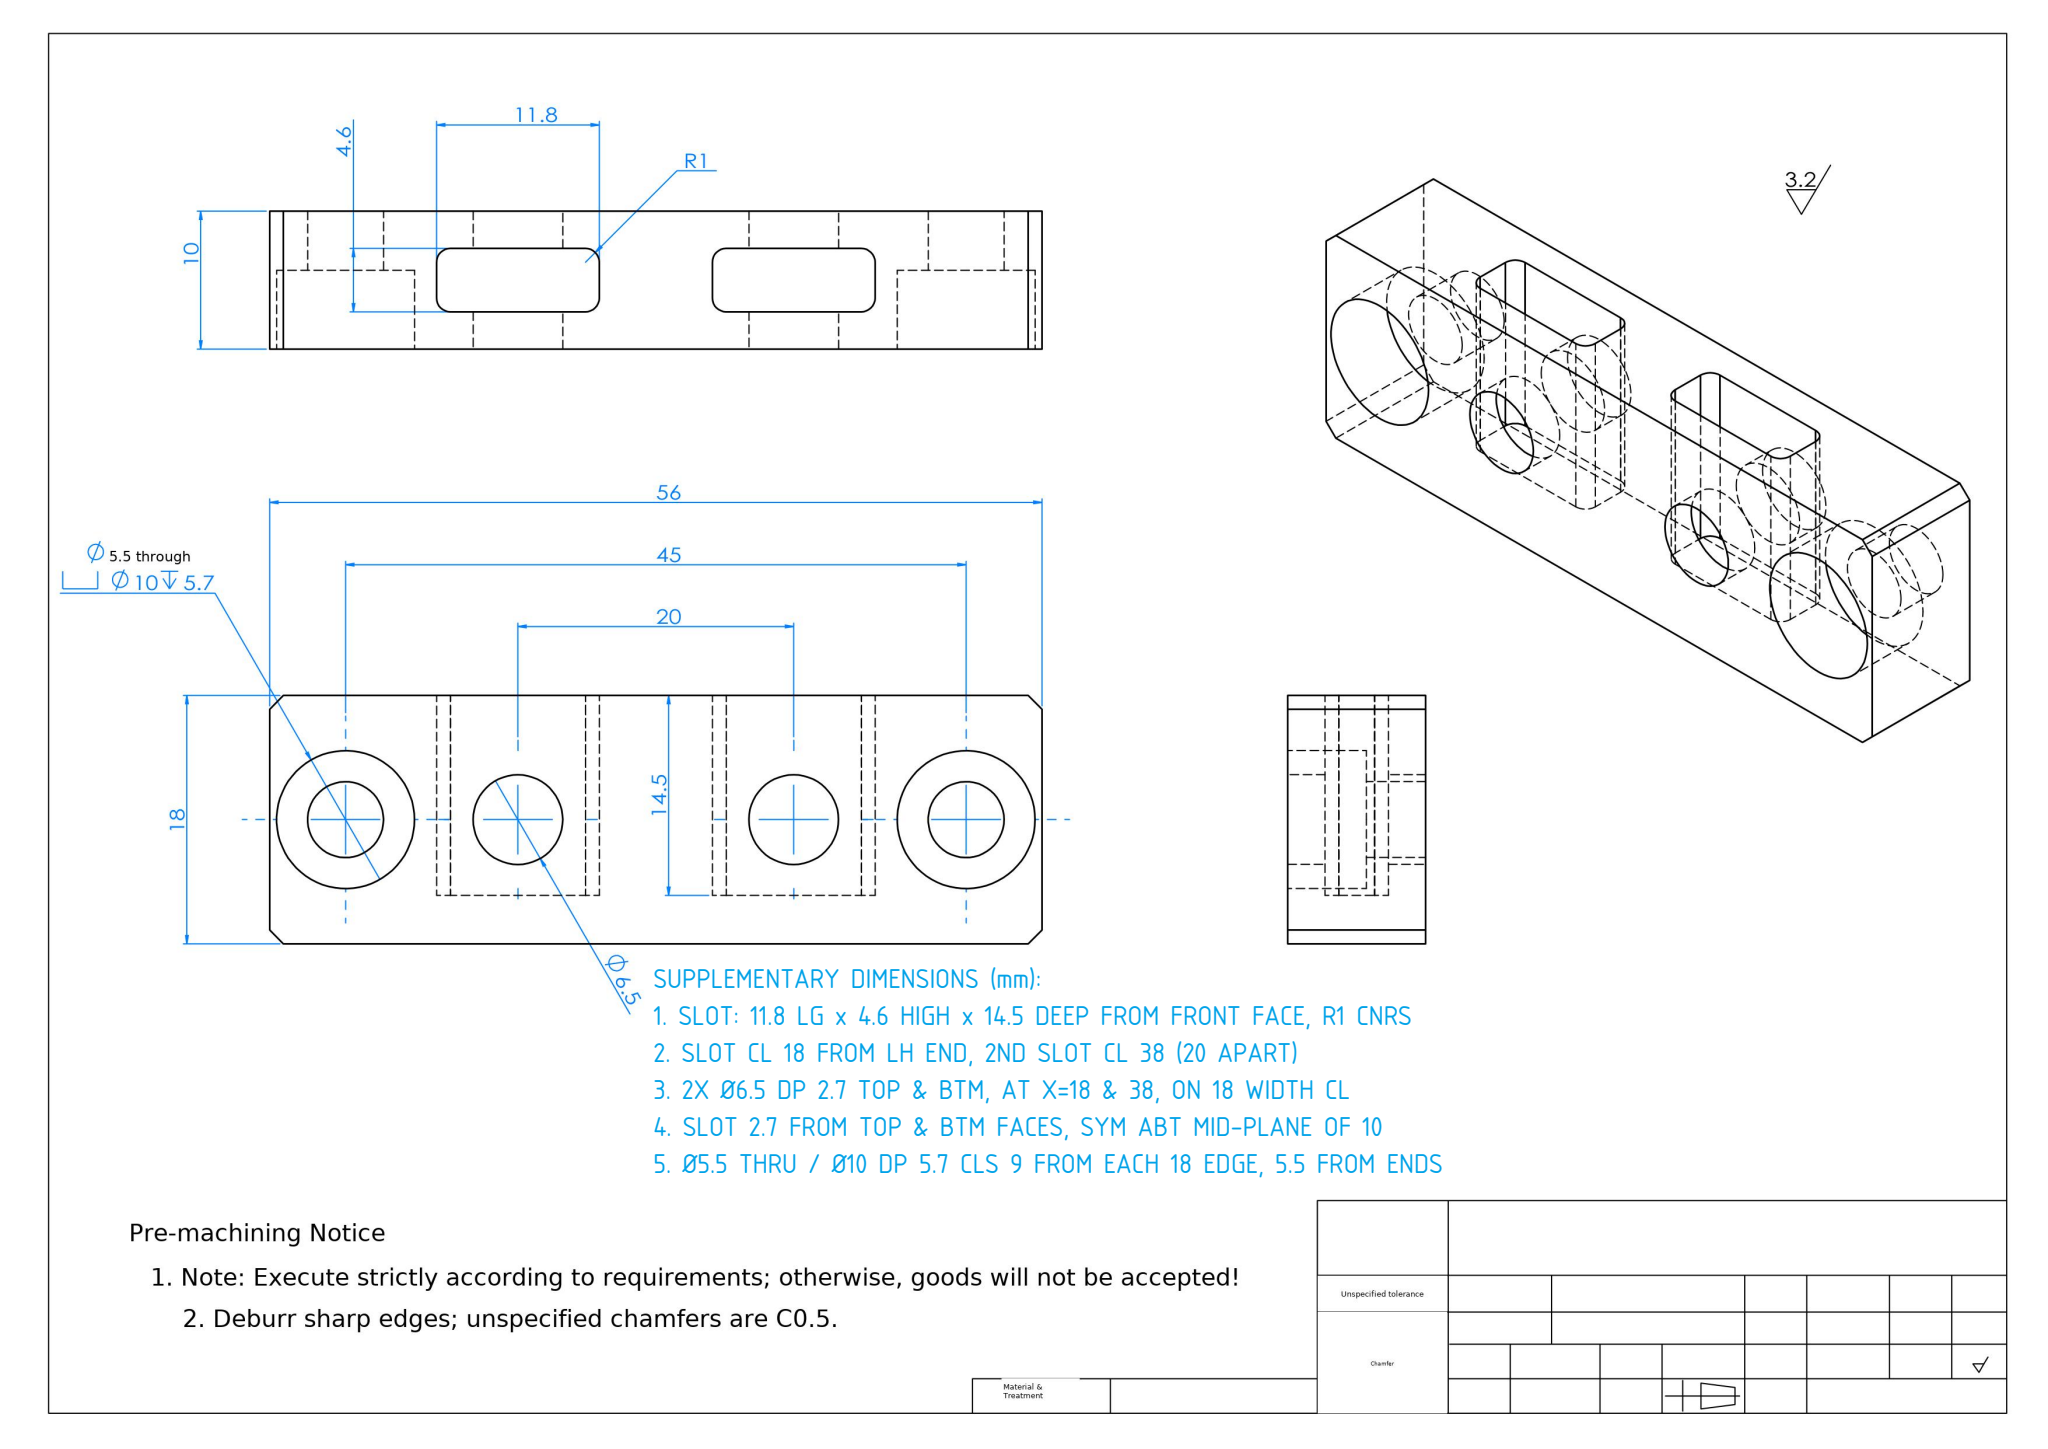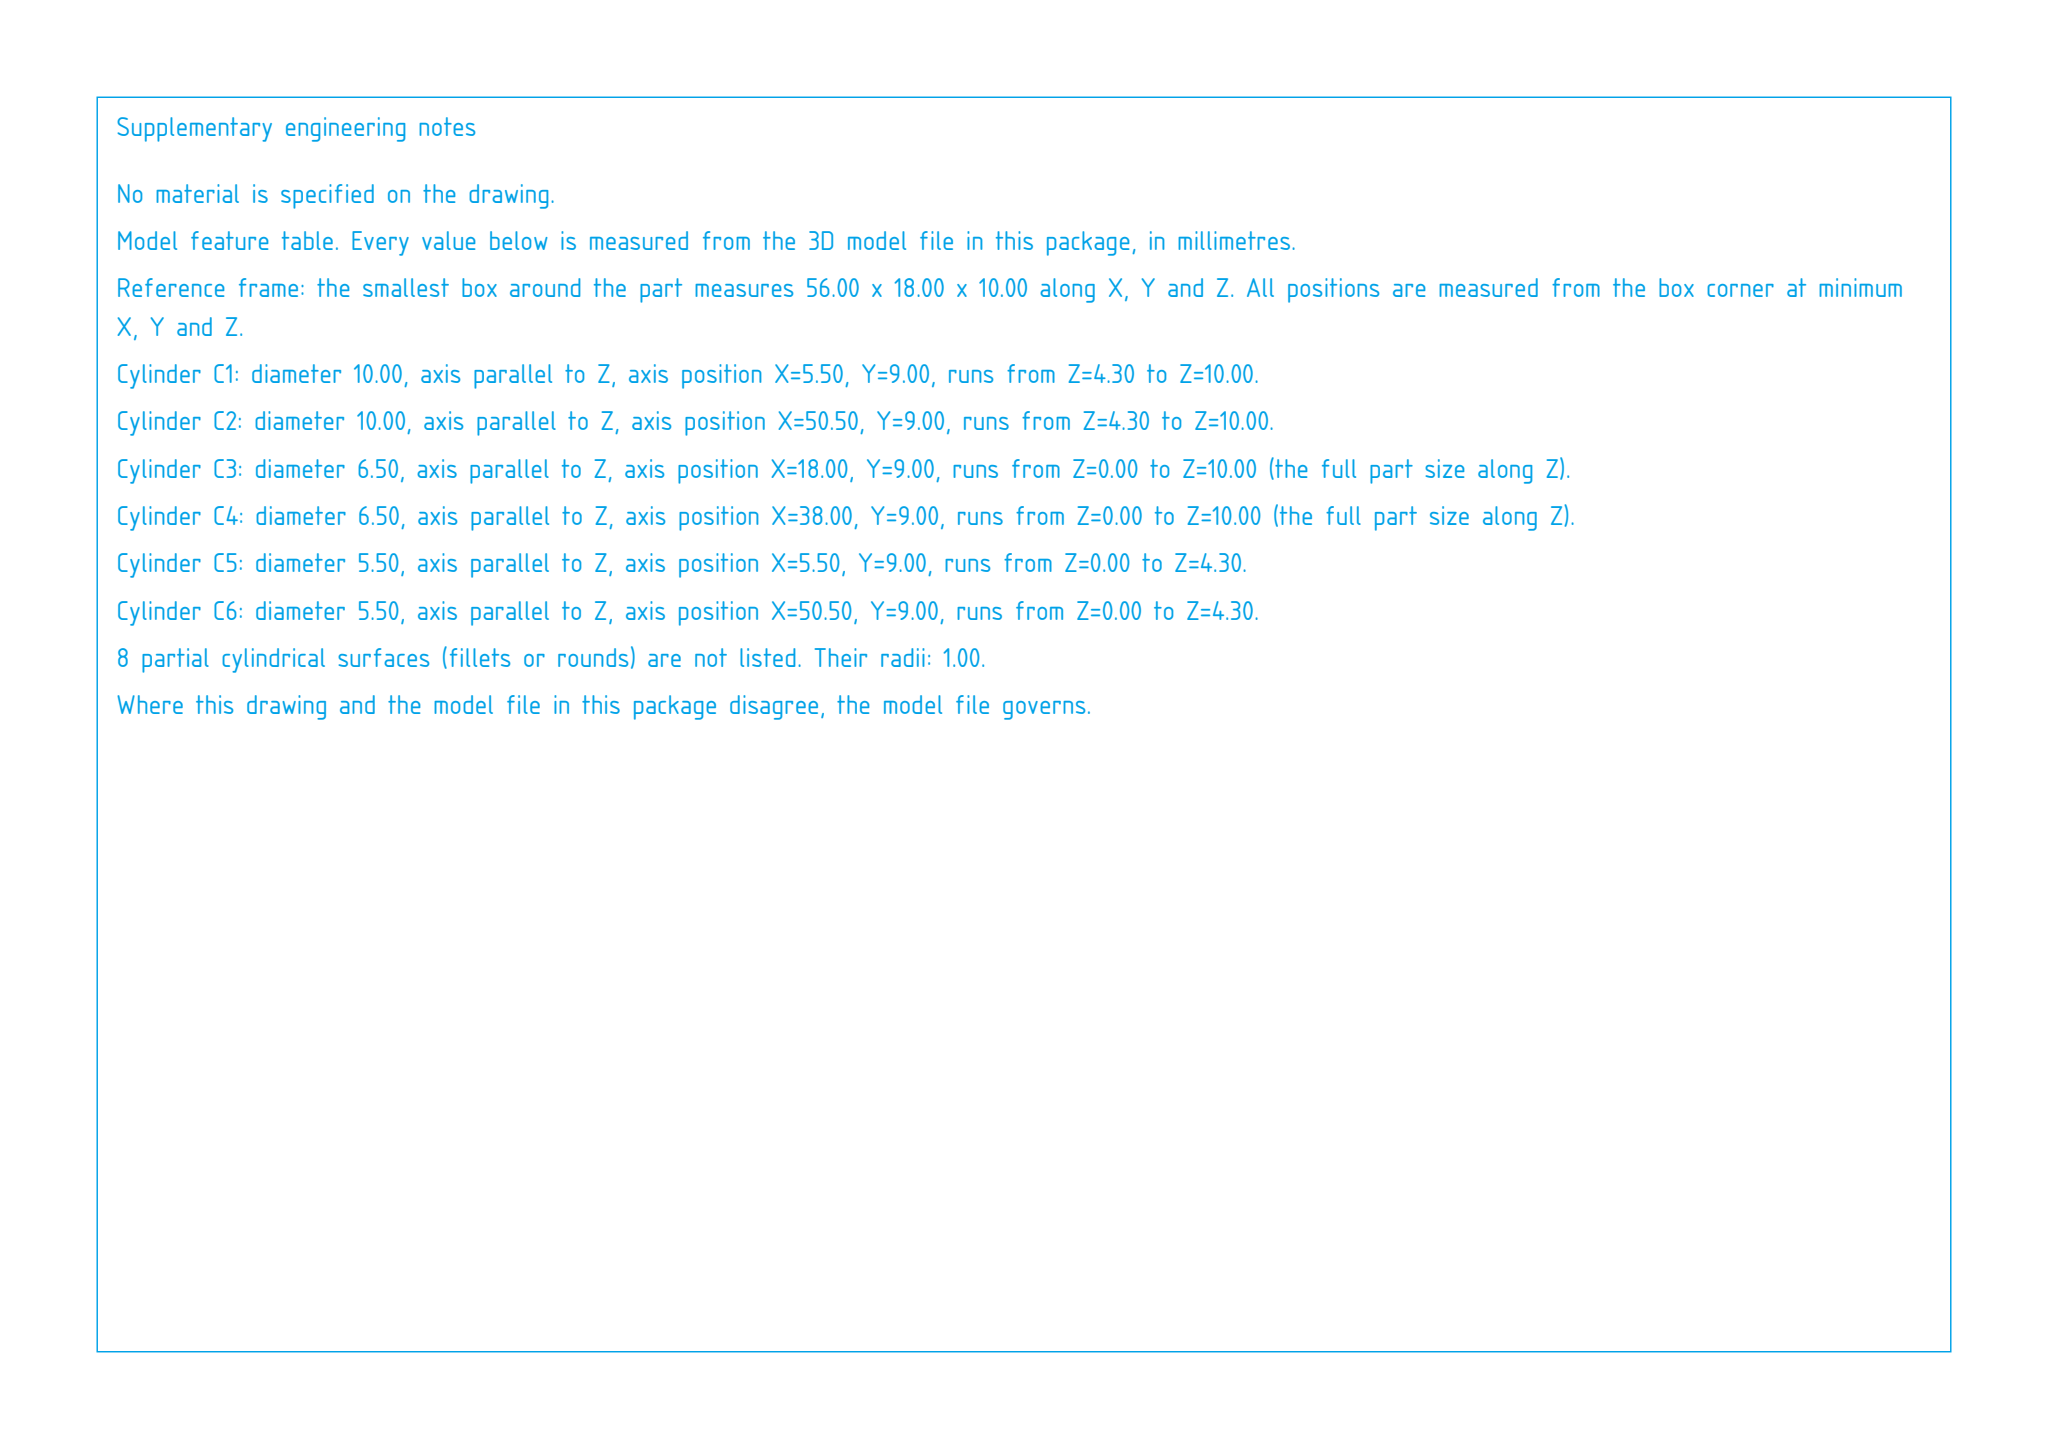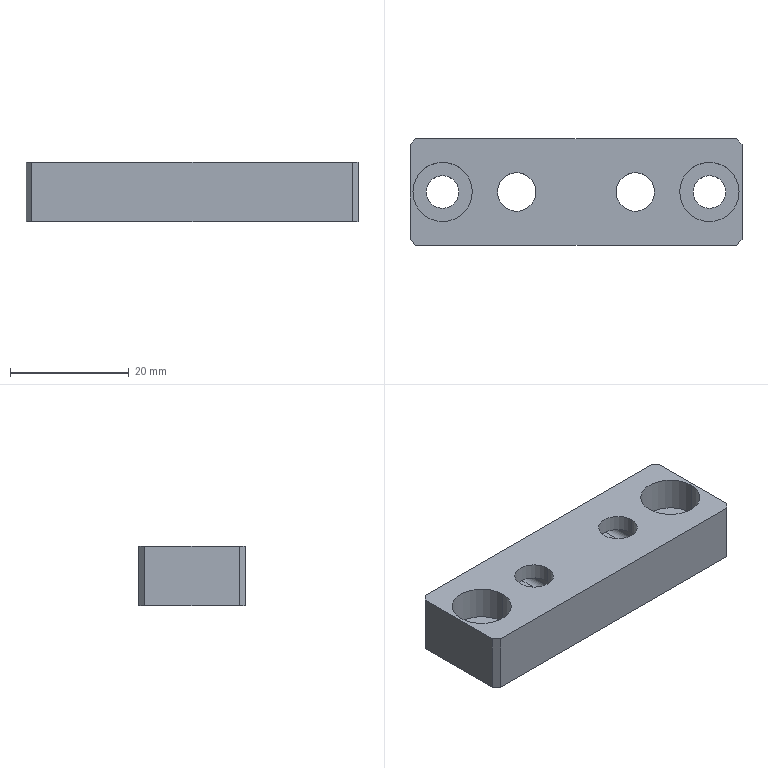Part | SolidWorks | mm | 1 solid | 46 faces | box 56 x 18 x 10 mm | volume 7053 mm3 | cylinder 24 | plane 22 | commonest cylinder face diameters 6.5 x8 2 x8 10 x4 5.5 x4
build123d program:
from build123d import *

# Parameters (mm, degrees)
SKETCH1_W                                            = 56
SKETCH1_H                                            = 18
BOSS_EXTRUDE1_DEPTH                                  = 10
CHAMFER1_SIZE                                        = 1
SKETCH2_W                                            = 11.8
SKETCH2_H                                            = 4.6
CUT_EXTRUDE1_DEPTH                                   = 14.5
F_6_5_6_5_DIAMETER_HOLE1_D                           = 6.5
F_6_5_6_5_DIAMETER_HOLE1_DEPTH                       = 12.4
F_6_5_6_5_DIAMETER_HOLE1_TIP                         = 1.953
HOLE_SIZE_ACCORDING_TO_HEXAGON_SOCKET_HE_D           = 5.5
HOLE_SIZE_ACCORDING_TO_HEXAGON_SOCKET_HE_CBORE_D     = 10
HOLE_SIZE_ACCORDING_TO_HEXAGON_SOCKET_HE_CBORE_DEPTH = 5.7
FILLET1_R                                            = 1


with BuildPart() as part:
    # Sketch1 → Boss-Extrude1 (new body)
    with BuildSketch(Plane.XY):
        Rectangle(SKETCH1_W, SKETCH1_H)
    extrude(amount=BOSS_EXTRUDE1_DEPTH)

    # Chamfer1
    chamfer1_edges = [part.edges().sort_by_distance(p)[0] for p in [
        (28, -9, 5),
        (-28, -9, 5),
        (-28, 9, 5),
        (28, 9, 5),
    ]]
    chamfer(chamfer1_edges, length=CHAMFER1_SIZE)

    # Sketch2 → Cut-Extrude1 (cut)
    with BuildSketch(Plane(origin=(0, 9, 0), x_dir=(1, 0, 0), z_dir=(0, 1, 0))):
        with Locations((-10, -5)):
            Rectangle(SKETCH2_W, SKETCH2_H)
        with Locations((10, -5)):
            Rectangle(SKETCH2_W, SKETCH2_H)
    extrude(amount=-CUT_EXTRUDE1_DEPTH, mode=Mode.SUBTRACT)

    # 6.5 _6.5_ Diameter Hole1
    with Locations(Plane.XY.offset(10)):
        with Locations((-10, 0), (10, 0)):
            Hole(F_6_5_6_5_DIAMETER_HOLE1_D / 2, depth=F_6_5_6_5_DIAMETER_HOLE1_DEPTH)
            with Locations((0, 0, -(F_6_5_6_5_DIAMETER_HOLE1_DEPTH + F_6_5_6_5_DIAMETER_HOLE1_TIP / 2))):  # 118° drill point
                Cone(0, F_6_5_6_5_DIAMETER_HOLE1_D / 2, F_6_5_6_5_DIAMETER_HOLE1_TIP, mode=Mode.SUBTRACT)

    # Hole Size_According to_Hexagon Socket He (through all)
    with Locations(Plane.XY.offset(10)):
        with Locations((-22.5, 0), (22.5, 0)):
            CounterBoreHole(HOLE_SIZE_ACCORDING_TO_HEXAGON_SOCKET_HE_D / 2, HOLE_SIZE_ACCORDING_TO_HEXAGON_SOCKET_HE_CBORE_D / 2, HOLE_SIZE_ACCORDING_TO_HEXAGON_SOCKET_HE_CBORE_DEPTH)

    # Fillet1
    fillet1_edges = [part.edges().sort_by_distance(p)[0] for p in [
        (-15.9, 1.75, 7.3),
        (-15.9, 1.75, 2.7),
        (-4.1, 1.75, 2.7),
        (-4.1, 1.75, 7.3),
        (4.1, 1.75, 2.7),
        (15.9, 1.75, 2.7),
        (15.9, 1.75, 7.3),
        (4.1, 1.75, 7.3),
    ]]
    fillet(fillet1_edges, radius=FILLET1_R)


solid = part.part